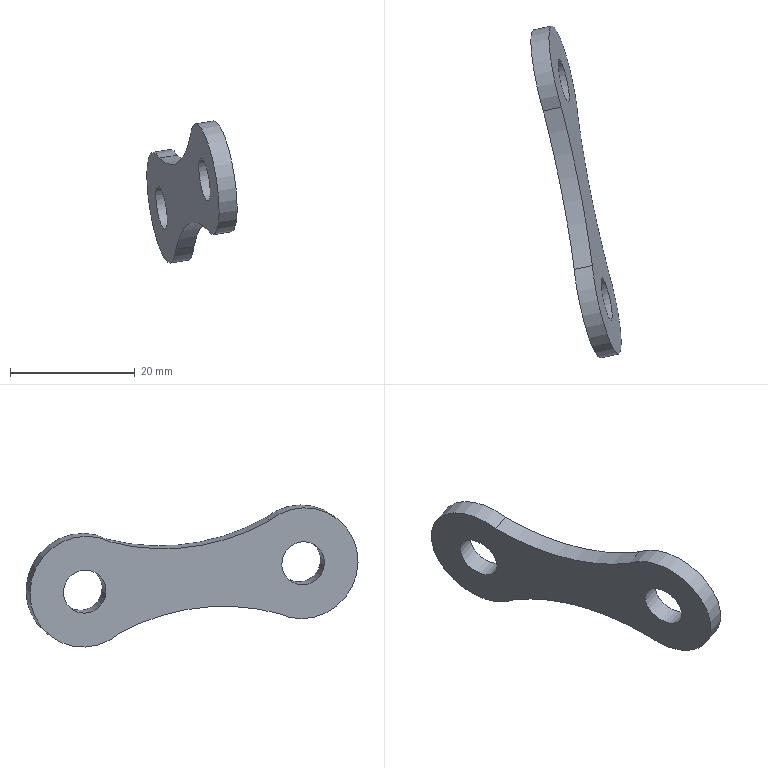Component | NX | 3_12 | 1 solid | 8 faces | box 14.49 x 53.27 x 22.8 mm | volume 1951 mm3 | cylinder 6 | plane 2 | commonest cylinder face diameters 70.075 x2 18 x2 7 x2
STEP:
#1=CARTESIAN_POINT('',(0.,0.,0.));
#2=DIRECTION('',(0.,0.,1.));
#3=DIRECTION('',(1.,0.,0.));
#4=AXIS2_PLACEMENT_3D('',#1,#2,#3);
#5=CARTESIAN_POINT('',(72.065,416.446,-165.474));
#6=VERTEX_POINT('',#5);
#7=CARTESIAN_POINT('',(74.96,417.076,-165.008));
#8=VERTEX_POINT('',#7);
#9=CARTESIAN_POINT('',(72.065,416.446,-165.474));
#10=DIRECTION('',(0.9653,0.21,0.1554));
#11=VECTOR('',#10,1.);
#12=LINE('',#9,#11);
#13=CARTESIAN_POINT('',(80.328,400.875,-195.754));
#14=DIRECTION('',(0.9653,0.21,0.1554));
#15=DIRECTION('',(0.1779,-0.09244,-0.9797));
#16=AXIS2_PLACEMENT_3D('',#13,#14,#15);
#17=CYLINDRICAL_SURFACE('',#16,35.038);
#18=CARTESIAN_POINT('',(2.764,-0.));
#19=DIRECTION('',(-0.,1.));
#20=VECTOR('',#19,1.);
#21=LINE('',#18,#20);
#22=(GEOMETRIC_REPRESENTATION_CONTEXT(2)PARAMETRIC_REPRESENTATION_CONTEXT()REPRESENTATION_CONTEXT('',''));
#23=DEFINITIONAL_REPRESENTATION('',(#21),#22);
#24=PCURVE('',#17,#23);
#25=CARTESIAN_POINT('',(69.774,422.032,-158.8));
#26=DIRECTION('',(0.9653,0.21,0.1554));
#27=DIRECTION('',(0.1779,-0.09244,-0.9797));
#28=AXIS2_PLACEMENT_3D('',#25,#26,#27);
#29=CYLINDRICAL_SURFACE('',#28,9.);
#30=CARTESIAN_POINT('',(-0.5931,-0.));
#31=DIRECTION('',(0.,1.));
#32=VECTOR('',#31,1.);
#33=LINE('',#30,#32);
#34=(GEOMETRIC_REPRESENTATION_CONTEXT(2)PARAMETRIC_REPRESENTATION_CONTEXT()REPRESENTATION_CONTEXT('',''));
#35=DEFINITIONAL_REPRESENTATION('',(#33),#34);
#36=PCURVE('',#29,#35);
#37=SURFACE_CURVE('',#12,(#24,#36),.PCURVE_S1.);
#38=EDGE_CURVE('',#6,#8,#37,.T.);
#39=ORIENTED_EDGE('',*,*,#38,.F.);
#40=CARTESIAN_POINT('',(77.093,390.984,-162.298));
#41=VERTEX_POINT('',#40);
#42=CARTESIAN_POINT('',(80.328,400.875,-195.754));
#43=DIRECTION('',(-0.9653,-0.21,-0.1554));
#44=DIRECTION('',(-0.1914,0.9733,-0.1266));
#45=AXIS2_PLACEMENT_3D('',#42,#43,#44);
#46=CIRCLE('',#45,35.038);
#47=CARTESIAN_POINT('',(7.854,0.));
#48=DIRECTION('',(-1.,-0.));
#49=VECTOR('',#48,1.);
#50=LINE('',#47,#49);
#51=(GEOMETRIC_REPRESENTATION_CONTEXT(2)PARAMETRIC_REPRESENTATION_CONTEXT()REPRESENTATION_CONTEXT('',''));
#52=DEFINITIONAL_REPRESENTATION('',(#50),#51);
#53=PCURVE('',#17,#52);
#54=CARTESIAN_POINT('',(75.051,411.454,-177.277));
#55=DIRECTION('',(-0.9653,-0.21,-0.1554));
#56=DIRECTION('',(-0.1779,0.09244,0.9797));
#57=AXIS2_PLACEMENT_3D('',#54,#55,#56);
#58=PLANE('',#57);
#59=CARTESIAN_POINT('',(-20.019,-8.967));
#60=DIRECTION('',(-0.,1.));
#61=AXIS2_PLACEMENT_2D('',#59,#60);
#62=CIRCLE('',#61,35.038);
#63=(GEOMETRIC_REPRESENTATION_CONTEXT(2)PARAMETRIC_REPRESENTATION_CONTEXT()REPRESENTATION_CONTEXT('',''));
#64=DEFINITIONAL_REPRESENTATION('',(#62),#63);
#65=PCURVE('',#58,#64);
#66=SURFACE_CURVE('',#46,(#53,#65),.PCURVE_S1.);
#67=EDGE_CURVE('',#41,#6,#66,.T.);
#68=ORIENTED_EDGE('',*,*,#67,.F.);
#69=CARTESIAN_POINT('',(79.988,391.614,-161.832));
#70=VERTEX_POINT('',#69);
#71=CARTESIAN_POINT('',(77.093,390.984,-162.298));
#72=DIRECTION('',(0.9653,0.21,0.1554));
#73=VECTOR('',#72,1.);
#74=LINE('',#71,#73);
#75=CARTESIAN_POINT('',(3.529,-0.));
#76=DIRECTION('',(0.,1.));
#77=VECTOR('',#76,1.);
#78=LINE('',#75,#77);
#79=(GEOMETRIC_REPRESENTATION_CONTEXT(2)PARAMETRIC_REPRESENTATION_CONTEXT()REPRESENTATION_CONTEXT('',''));
#80=DEFINITIONAL_REPRESENTATION('',(#78),#79);
#81=PCURVE('',#17,#80);
#82=CARTESIAN_POINT('',(76.664,386.993,-154.243));
#83=DIRECTION('',(0.9653,0.21,0.1554));
#84=DIRECTION('',(0.1779,-0.09244,-0.9797));
#85=AXIS2_PLACEMENT_3D('',#82,#83,#84);
#86=CYLINDRICAL_SURFACE('',#85,9.);
#87=CARTESIAN_POINT('',(6.849,-0.));
#88=DIRECTION('',(0.,1.));
#89=VECTOR('',#88,1.);
#90=LINE('',#87,#89);
#91=(GEOMETRIC_REPRESENTATION_CONTEXT(2)PARAMETRIC_REPRESENTATION_CONTEXT()REPRESENTATION_CONTEXT('',''));
#92=DEFINITIONAL_REPRESENTATION('',(#90),#91);
#93=PCURVE('',#86,#92);
#94=SURFACE_CURVE('',#74,(#81,#93),.PCURVE_S1.);
#95=EDGE_CURVE('',#41,#70,#94,.T.);
#96=ORIENTED_EDGE('',*,*,#95,.T.);
#97=CARTESIAN_POINT('',(83.224,401.505,-195.288));
#98=DIRECTION('',(-0.9653,-0.21,-0.1554));
#99=DIRECTION('',(-0.1914,0.9733,-0.1266));
#100=AXIS2_PLACEMENT_3D('',#97,#98,#99);
#101=CIRCLE('',#100,35.038);
#102=CARTESIAN_POINT('',(7.854,3.));
#103=DIRECTION('',(-1.,0.));
#104=VECTOR('',#103,1.);
#105=LINE('',#102,#104);
#106=(GEOMETRIC_REPRESENTATION_CONTEXT(2)PARAMETRIC_REPRESENTATION_CONTEXT()REPRESENTATION_CONTEXT('',''));
#107=DEFINITIONAL_REPRESENTATION('',(#105),#106);
#108=PCURVE('',#17,#107);
#109=CARTESIAN_POINT('',(77.947,412.084,-176.811));
#110=DIRECTION('',(-0.9653,-0.21,-0.1554));
#111=DIRECTION('',(-0.1779,0.09244,0.9797));
#112=AXIS2_PLACEMENT_3D('',#109,#110,#111);
#113=PLANE('',#112);
#114=CARTESIAN_POINT('',(-20.019,-8.967));
#115=DIRECTION('',(-0.,1.));
#116=AXIS2_PLACEMENT_2D('',#114,#115);
#117=CIRCLE('',#116,35.038);
#118=(GEOMETRIC_REPRESENTATION_CONTEXT(2)PARAMETRIC_REPRESENTATION_CONTEXT()REPRESENTATION_CONTEXT('',''));
#119=DEFINITIONAL_REPRESENTATION('',(#117),#118);
#120=PCURVE('',#113,#119);
#121=SURFACE_CURVE('',#101,(#108,#120),.PCURVE_S1.);
#122=EDGE_CURVE('',#70,#8,#121,.T.);
#123=ORIENTED_EDGE('',*,*,#122,.T.);
#124=EDGE_LOOP('',(#39,#68,#96,#123));
#125=FACE_BOUND('',#124,.F.);
#126=ADVANCED_FACE('',(#125),#17,.F.);
#127=CARTESIAN_POINT('',(72.306,418.456,-150.385));
#128=VERTEX_POINT('',#127);
#129=CARTESIAN_POINT('',(72.67,422.662,-158.333));
#130=DIRECTION('',(0.9653,0.21,0.1554));
#131=DIRECTION('',(-0.1914,0.9733,-0.1266));
#132=AXIS2_PLACEMENT_3D('',#129,#130,#131);
#133=CIRCLE('',#132,9.);
#134=CARTESIAN_POINT('',(-4.712,3.));
#135=DIRECTION('',(1.,0.));
#136=VECTOR('',#135,1.);
#137=LINE('',#134,#136);
#138=(GEOMETRIC_REPRESENTATION_CONTEXT(2)PARAMETRIC_REPRESENTATION_CONTEXT()REPRESENTATION_CONTEXT('',''));
#139=DEFINITIONAL_REPRESENTATION('',(#137),#138);
#140=PCURVE('',#29,#139);
#141=CARTESIAN_POINT('',(20.019,17.967));
#142=CARTESIAN_POINT('',(35.607,17.967));
#143=CARTESIAN_POINT('',(27.813,4.467));
#144=CARTESIAN_POINT('',(20.019,-9.033));
#145=CARTESIAN_POINT('',(12.225,4.467));
#146=CARTESIAN_POINT('',(4.43,17.967));
#147=CARTESIAN_POINT('',(20.019,17.967));
#148=(BOUNDED_CURVE()B_SPLINE_CURVE(2,(#141,#142,#143,#144,#145,#146,#147),.UNSPECIFIED.,.T.,.F.)B_SPLINE_CURVE_WITH_KNOTS((1,2,2,2,2,1),(-2.094,0.,2.094,4.189,6.283,8.378),.UNSPECIFIED.)CURVE()GEOMETRIC_REPRESENTATION_ITEM()RATIONAL_B_SPLINE_CURVE((1.,0.5,1.,0.5,1.,0.5,1.))REPRESENTATION_ITEM(''));
#149=(GEOMETRIC_REPRESENTATION_CONTEXT(2)PARAMETRIC_REPRESENTATION_CONTEXT()REPRESENTATION_CONTEXT('',''));
#150=DEFINITIONAL_REPRESENTATION('',(#148),#149);
#151=PCURVE('',#113,#150);
#152=SURFACE_CURVE('',#133,(#140,#151),.PCURVE_S1.);
#153=EDGE_CURVE('',#8,#128,#152,.T.);
#154=ORIENTED_EDGE('',*,*,#153,.F.);
#155=ORIENTED_EDGE('',*,*,#38,.F.);
#156=CARTESIAN_POINT('',(69.41,417.826,-150.852));
#157=VERTEX_POINT('',#156);
#158=CARTESIAN_POINT('',(69.774,422.032,-158.8));
#159=DIRECTION('',(0.9653,0.21,0.1554));
#160=DIRECTION('',(-0.1914,0.9733,-0.1266));
#161=AXIS2_PLACEMENT_3D('',#158,#159,#160);
#162=CIRCLE('',#161,9.);
#163=CARTESIAN_POINT('',(-4.712,-0.));
#164=DIRECTION('',(1.,0.));
#165=VECTOR('',#164,1.);
#166=LINE('',#163,#165);
#167=(GEOMETRIC_REPRESENTATION_CONTEXT(2)PARAMETRIC_REPRESENTATION_CONTEXT()REPRESENTATION_CONTEXT('',''));
#168=DEFINITIONAL_REPRESENTATION('',(#166),#167);
#169=PCURVE('',#29,#168);
#170=CARTESIAN_POINT('',(20.019,17.967));
#171=CARTESIAN_POINT('',(35.607,17.967));
#172=CARTESIAN_POINT('',(27.813,4.467));
#173=CARTESIAN_POINT('',(20.019,-9.033));
#174=CARTESIAN_POINT('',(12.225,4.467));
#175=CARTESIAN_POINT('',(4.43,17.967));
#176=CARTESIAN_POINT('',(20.019,17.967));
#177=(BOUNDED_CURVE()B_SPLINE_CURVE(2,(#170,#171,#172,#173,#174,#175,#176),.UNSPECIFIED.,.T.,.F.)B_SPLINE_CURVE_WITH_KNOTS((1,2,2,2,2,1),(-2.094,0.,2.094,4.189,6.283,8.378),.UNSPECIFIED.)CURVE()GEOMETRIC_REPRESENTATION_ITEM()RATIONAL_B_SPLINE_CURVE((1.,0.5,1.,0.5,1.,0.5,1.))REPRESENTATION_ITEM(''));
#178=(GEOMETRIC_REPRESENTATION_CONTEXT(2)PARAMETRIC_REPRESENTATION_CONTEXT()REPRESENTATION_CONTEXT('',''));
#179=DEFINITIONAL_REPRESENTATION('',(#177),#178);
#180=PCURVE('',#58,#179);
#181=SURFACE_CURVE('',#162,(#169,#180),.PCURVE_S1.);
#182=EDGE_CURVE('',#6,#157,#181,.T.);
#183=ORIENTED_EDGE('',*,*,#182,.T.);
#184=CARTESIAN_POINT('',(69.41,417.826,-150.852));
#185=DIRECTION('',(0.9653,0.21,0.1554));
#186=VECTOR('',#185,1.);
#187=LINE('',#184,#186);
#188=CARTESIAN_POINT('',(3.735,0.));
#189=DIRECTION('',(-0.,1.));
#190=VECTOR('',#189,1.);
#191=LINE('',#188,#190);
#192=(GEOMETRIC_REPRESENTATION_CONTEXT(2)PARAMETRIC_REPRESENTATION_CONTEXT()REPRESENTATION_CONTEXT('',''));
#193=DEFINITIONAL_REPRESENTATION('',(#191),#192);
#194=PCURVE('',#29,#193);
#195=CARTESIAN_POINT('',(66.085,408.277,-117.305));
#196=DIRECTION('',(0.9653,0.21,0.1554));
#197=DIRECTION('',(0.1779,-0.09244,-0.9797));
#198=AXIS2_PLACEMENT_3D('',#195,#196,#197);
#199=CYLINDRICAL_SURFACE('',#198,35.038);
#200=CARTESIAN_POINT('',(6.66,0.));
#201=DIRECTION('',(0.,1.));
#202=VECTOR('',#201,1.);
#203=LINE('',#200,#202);
#204=(GEOMETRIC_REPRESENTATION_CONTEXT(2)PARAMETRIC_REPRESENTATION_CONTEXT()REPRESENTATION_CONTEXT('',''));
#205=DEFINITIONAL_REPRESENTATION('',(#203),#204);
#206=PCURVE('',#199,#205);
#207=SURFACE_CURVE('',#187,(#194,#206),.PCURVE_S1.);
#208=EDGE_CURVE('',#157,#128,#207,.T.);
#209=ORIENTED_EDGE('',*,*,#208,.T.);
#210=EDGE_LOOP('',(#154,#155,#183,#209));
#211=FACE_BOUND('',#210,.T.);
#212=ADVANCED_FACE('',(#211),#29,.T.);
#213=CARTESIAN_POINT('',(74.389,392.389,-147.408));
#214=VERTEX_POINT('',#213);
#215=CARTESIAN_POINT('',(77.285,393.019,-146.942));
#216=VERTEX_POINT('',#215);
#217=CARTESIAN_POINT('',(74.389,392.389,-147.408));
#218=DIRECTION('',(0.9653,0.21,0.1554));
#219=VECTOR('',#218,1.);
#220=LINE('',#217,#219);
#221=CARTESIAN_POINT('',(5.896,0.));
#222=DIRECTION('',(0.,1.));
#223=VECTOR('',#222,1.);
#224=LINE('',#221,#223);
#225=(GEOMETRIC_REPRESENTATION_CONTEXT(2)PARAMETRIC_REPRESENTATION_CONTEXT()REPRESENTATION_CONTEXT('',''));
#226=DEFINITIONAL_REPRESENTATION('',(#224),#225);
#227=PCURVE('',#199,#226);
#228=CARTESIAN_POINT('',(2.576,-0.));
#229=DIRECTION('',(0.,1.));
#230=VECTOR('',#229,1.);
#231=LINE('',#228,#230);
#232=(GEOMETRIC_REPRESENTATION_CONTEXT(2)PARAMETRIC_REPRESENTATION_CONTEXT()REPRESENTATION_CONTEXT('',''));
#233=DEFINITIONAL_REPRESENTATION('',(#231),#232);
#234=PCURVE('',#86,#233);
#235=SURFACE_CURVE('',#220,(#227,#234),.PCURVE_S1.);
#236=EDGE_CURVE('',#214,#216,#235,.T.);
#237=ORIENTED_EDGE('',*,*,#236,.F.);
#238=CARTESIAN_POINT('',(66.085,408.277,-117.305));
#239=DIRECTION('',(-0.9653,-0.21,-0.1554));
#240=DIRECTION('',(-0.1914,0.9733,-0.1266));
#241=AXIS2_PLACEMENT_3D('',#238,#239,#240);
#242=CIRCLE('',#241,35.038);
#243=CARTESIAN_POINT('',(7.854,0.));
#244=DIRECTION('',(-1.,0.));
#245=VECTOR('',#244,1.);
#246=LINE('',#243,#245);
#247=(GEOMETRIC_REPRESENTATION_CONTEXT(2)PARAMETRIC_REPRESENTATION_CONTEXT()REPRESENTATION_CONTEXT('',''));
#248=DEFINITIONAL_REPRESENTATION('',(#246),#247);
#249=PCURVE('',#199,#248);
#250=CARTESIAN_POINT('',(60.056,-8.967));
#251=DIRECTION('',(-0.,1.));
#252=AXIS2_PLACEMENT_2D('',#250,#251);
#253=CIRCLE('',#252,35.038);
#254=(GEOMETRIC_REPRESENTATION_CONTEXT(2)PARAMETRIC_REPRESENTATION_CONTEXT()REPRESENTATION_CONTEXT('',''));
#255=DEFINITIONAL_REPRESENTATION('',(#253),#254);
#256=PCURVE('',#58,#255);
#257=SURFACE_CURVE('',#242,(#249,#256),.PCURVE_S1.);
#258=EDGE_CURVE('',#157,#214,#257,.T.);
#259=ORIENTED_EDGE('',*,*,#258,.F.);
#260=ORIENTED_EDGE('',*,*,#208,.T.);
#261=CARTESIAN_POINT('',(68.981,408.907,-116.838));
#262=DIRECTION('',(-0.9653,-0.21,-0.1554));
#263=DIRECTION('',(-0.1914,0.9733,-0.1266));
#264=AXIS2_PLACEMENT_3D('',#261,#262,#263);
#265=CIRCLE('',#264,35.038);
#266=CARTESIAN_POINT('',(7.854,3.));
#267=DIRECTION('',(-1.,0.));
#268=VECTOR('',#267,1.);
#269=LINE('',#266,#268);
#270=(GEOMETRIC_REPRESENTATION_CONTEXT(2)PARAMETRIC_REPRESENTATION_CONTEXT()REPRESENTATION_CONTEXT('',''));
#271=DEFINITIONAL_REPRESENTATION('',(#269),#270);
#272=PCURVE('',#199,#271);
#273=CARTESIAN_POINT('',(60.056,-8.967));
#274=DIRECTION('',(-0.,1.));
#275=AXIS2_PLACEMENT_2D('',#273,#274);
#276=CIRCLE('',#275,35.038);
#277=(GEOMETRIC_REPRESENTATION_CONTEXT(2)PARAMETRIC_REPRESENTATION_CONTEXT()REPRESENTATION_CONTEXT('',''));
#278=DEFINITIONAL_REPRESENTATION('',(#276),#277);
#279=PCURVE('',#113,#278);
#280=SURFACE_CURVE('',#265,(#272,#279),.PCURVE_S1.);
#281=EDGE_CURVE('',#128,#216,#280,.T.);
#282=ORIENTED_EDGE('',*,*,#281,.T.);
#283=EDGE_LOOP('',(#237,#259,#260,#282));
#284=FACE_BOUND('',#283,.F.);
#285=ADVANCED_FACE('',(#284),#199,.F.);
#286=CARTESIAN_POINT('',(75.994,390.399,-154.686));
#287=VERTEX_POINT('',#286);
#288=CARTESIAN_POINT('',(76.664,386.993,-154.243));
#289=DIRECTION('',(0.9653,0.21,0.1554));
#290=DIRECTION('',(-0.1914,0.9733,-0.1266));
#291=AXIS2_PLACEMENT_3D('',#288,#289,#290);
#292=CIRCLE('',#291,3.5);
#293=CARTESIAN_POINT('',(76.664,386.993,-154.243));
#294=DIRECTION('',(0.9653,0.21,0.1554));
#295=DIRECTION('',(0.1779,-0.09244,-0.9797));
#296=AXIS2_PLACEMENT_3D('',#293,#294,#295);
#297=CYLINDRICAL_SURFACE('',#296,3.5);
#298=CARTESIAN_POINT('',(1.571,0.));
#299=DIRECTION('',(1.,0.));
#300=VECTOR('',#299,1.);
#301=LINE('',#298,#300);
#302=(GEOMETRIC_REPRESENTATION_CONTEXT(2)PARAMETRIC_REPRESENTATION_CONTEXT()REPRESENTATION_CONTEXT('',''));
#303=DEFINITIONAL_REPRESENTATION('',(#301),#302);
#304=PCURVE('',#297,#303);
#305=CARTESIAN_POINT('',(20.019,-23.533));
#306=CARTESIAN_POINT('',(26.081,-23.533));
#307=CARTESIAN_POINT('',(23.05,-28.783));
#308=CARTESIAN_POINT('',(20.019,-34.033));
#309=CARTESIAN_POINT('',(16.988,-28.783));
#310=CARTESIAN_POINT('',(13.957,-23.533));
#311=CARTESIAN_POINT('',(20.019,-23.533));
#312=(BOUNDED_CURVE()B_SPLINE_CURVE(2,(#305,#306,#307,#308,#309,#310,#311),.UNSPECIFIED.,.T.,.F.)B_SPLINE_CURVE_WITH_KNOTS((1,2,2,2,2,1),(-2.094,0.,2.094,4.189,6.283,8.378),.UNSPECIFIED.)CURVE()GEOMETRIC_REPRESENTATION_ITEM()RATIONAL_B_SPLINE_CURVE((1.,0.5,1.,0.5,1.,0.5,1.))REPRESENTATION_ITEM(''));
#313=(GEOMETRIC_REPRESENTATION_CONTEXT(2)PARAMETRIC_REPRESENTATION_CONTEXT()REPRESENTATION_CONTEXT('',''));
#314=DEFINITIONAL_REPRESENTATION('',(#312),#313);
#315=PCURVE('',#58,#314);
#316=SURFACE_CURVE('',#292,(#304,#315),.PCURVE_S1.);
#317=EDGE_CURVE('',#287,#287,#316,.T.);
#318=ORIENTED_EDGE('',*,*,#317,.T.);
#319=CARTESIAN_POINT('',(78.89,391.029,-154.219));
#320=VERTEX_POINT('',#319);
#321=CARTESIAN_POINT('',(75.994,390.399,-154.686));
#322=CARTESIAN_POINT('',(78.89,391.029,-154.219));
#323=B_SPLINE_CURVE_WITH_KNOTS('',1,(#321,#322),.UNSPECIFIED.,.F.,.F.,(2,2),(0.,3.),.PIECEWISE_BEZIER_KNOTS.);
#324=CARTESIAN_POINT('',(7.854,0.));
#325=DIRECTION('',(0.,1.));
#326=VECTOR('',#325,1.);
#327=LINE('',#324,#326);
#328=(GEOMETRIC_REPRESENTATION_CONTEXT(2)PARAMETRIC_REPRESENTATION_CONTEXT()REPRESENTATION_CONTEXT('',''));
#329=DEFINITIONAL_REPRESENTATION('',(#327),#328);
#330=PCURVE('',#297,#329);
#331=CARTESIAN_POINT('',(1.571,0.));
#332=DIRECTION('',(0.,1.));
#333=VECTOR('',#332,1.);
#334=LINE('',#331,#333);
#335=(GEOMETRIC_REPRESENTATION_CONTEXT(2)PARAMETRIC_REPRESENTATION_CONTEXT()REPRESENTATION_CONTEXT('',''));
#336=DEFINITIONAL_REPRESENTATION('',(#334),#335);
#337=PCURVE('',#297,#336);
#338=SEAM_CURVE('',#323,(#330,#337),.PCURVE_S1.);
#339=EDGE_CURVE('',#287,#320,#338,.T.);
#340=ORIENTED_EDGE('',*,*,#339,.T.);
#341=CARTESIAN_POINT('',(79.56,387.623,-153.776));
#342=DIRECTION('',(0.9653,0.21,0.1554));
#343=DIRECTION('',(-0.1914,0.9733,-0.1266));
#344=AXIS2_PLACEMENT_3D('',#341,#342,#343);
#345=CIRCLE('',#344,3.5);
#346=CARTESIAN_POINT('',(1.571,3.));
#347=DIRECTION('',(1.,0.));
#348=VECTOR('',#347,1.);
#349=LINE('',#346,#348);
#350=(GEOMETRIC_REPRESENTATION_CONTEXT(2)PARAMETRIC_REPRESENTATION_CONTEXT()REPRESENTATION_CONTEXT('',''));
#351=DEFINITIONAL_REPRESENTATION('',(#349),#350);
#352=PCURVE('',#297,#351);
#353=CARTESIAN_POINT('',(20.019,-23.533));
#354=CARTESIAN_POINT('',(26.081,-23.533));
#355=CARTESIAN_POINT('',(23.05,-28.783));
#356=CARTESIAN_POINT('',(20.019,-34.033));
#357=CARTESIAN_POINT('',(16.988,-28.783));
#358=CARTESIAN_POINT('',(13.957,-23.533));
#359=CARTESIAN_POINT('',(20.019,-23.533));
#360=(BOUNDED_CURVE()B_SPLINE_CURVE(2,(#353,#354,#355,#356,#357,#358,#359),.UNSPECIFIED.,.T.,.F.)B_SPLINE_CURVE_WITH_KNOTS((1,2,2,2,2,1),(-2.094,0.,2.094,4.189,6.283,8.378),.UNSPECIFIED.)CURVE()GEOMETRIC_REPRESENTATION_ITEM()RATIONAL_B_SPLINE_CURVE((1.,0.5,1.,0.5,1.,0.5,1.))REPRESENTATION_ITEM(''));
#361=(GEOMETRIC_REPRESENTATION_CONTEXT(2)PARAMETRIC_REPRESENTATION_CONTEXT()REPRESENTATION_CONTEXT('',''));
#362=DEFINITIONAL_REPRESENTATION('',(#360),#361);
#363=PCURVE('',#113,#362);
#364=SURFACE_CURVE('',#345,(#352,#363),.PCURVE_S1.);
#365=EDGE_CURVE('',#320,#320,#364,.T.);
#366=ORIENTED_EDGE('',*,*,#365,.F.);
#367=ORIENTED_EDGE('',*,*,#339,.F.);
#368=EDGE_LOOP('',(#318,#340,#366,#367));
#369=FACE_BOUND('',#368,.F.);
#370=ADVANCED_FACE('',(#369),#297,.F.);
#371=CARTESIAN_POINT('',(79.56,387.623,-153.776));
#372=DIRECTION('',(0.9653,0.21,0.1554));
#373=DIRECTION('',(-0.1914,0.9733,-0.1266));
#374=AXIS2_PLACEMENT_3D('',#371,#372,#373);
#375=CIRCLE('',#374,9.);
#376=CARTESIAN_POINT('',(1.571,3.));
#377=DIRECTION('',(1.,-0.));
#378=VECTOR('',#377,1.);
#379=LINE('',#376,#378);
#380=(GEOMETRIC_REPRESENTATION_CONTEXT(2)PARAMETRIC_REPRESENTATION_CONTEXT()REPRESENTATION_CONTEXT('',''));
#381=DEFINITIONAL_REPRESENTATION('',(#379),#380);
#382=PCURVE('',#86,#381);
#383=CARTESIAN_POINT('',(20.019,-18.033));
#384=CARTESIAN_POINT('',(35.607,-18.033));
#385=CARTESIAN_POINT('',(27.813,-31.533));
#386=CARTESIAN_POINT('',(20.019,-45.033));
#387=CARTESIAN_POINT('',(12.225,-31.533));
#388=CARTESIAN_POINT('',(4.43,-18.033));
#389=CARTESIAN_POINT('',(20.019,-18.033));
#390=(BOUNDED_CURVE()B_SPLINE_CURVE(2,(#383,#384,#385,#386,#387,#388,#389),.UNSPECIFIED.,.T.,.F.)B_SPLINE_CURVE_WITH_KNOTS((1,2,2,2,2,1),(-2.094,0.,2.094,4.189,6.283,8.378),.UNSPECIFIED.)CURVE()GEOMETRIC_REPRESENTATION_ITEM()RATIONAL_B_SPLINE_CURVE((1.,0.5,1.,0.5,1.,0.5,1.))REPRESENTATION_ITEM(''));
#391=(GEOMETRIC_REPRESENTATION_CONTEXT(2)PARAMETRIC_REPRESENTATION_CONTEXT()REPRESENTATION_CONTEXT('',''));
#392=DEFINITIONAL_REPRESENTATION('',(#390),#391);
#393=PCURVE('',#113,#392);
#394=SURFACE_CURVE('',#375,(#382,#393),.PCURVE_S1.);
#395=EDGE_CURVE('',#216,#70,#394,.T.);
#396=ORIENTED_EDGE('',*,*,#395,.F.);
#397=ORIENTED_EDGE('',*,*,#236,.F.);
#398=CARTESIAN_POINT('',(76.664,386.993,-154.243));
#399=DIRECTION('',(0.9653,0.21,0.1554));
#400=DIRECTION('',(-0.1914,0.9733,-0.1266));
#401=AXIS2_PLACEMENT_3D('',#398,#399,#400);
#402=CIRCLE('',#401,9.);
#403=CARTESIAN_POINT('',(1.571,-0.));
#404=DIRECTION('',(1.,0.));
#405=VECTOR('',#404,1.);
#406=LINE('',#403,#405);
#407=(GEOMETRIC_REPRESENTATION_CONTEXT(2)PARAMETRIC_REPRESENTATION_CONTEXT()REPRESENTATION_CONTEXT('',''));
#408=DEFINITIONAL_REPRESENTATION('',(#406),#407);
#409=PCURVE('',#86,#408);
#410=CARTESIAN_POINT('',(20.019,-18.033));
#411=CARTESIAN_POINT('',(35.607,-18.033));
#412=CARTESIAN_POINT('',(27.813,-31.533));
#413=CARTESIAN_POINT('',(20.019,-45.033));
#414=CARTESIAN_POINT('',(12.225,-31.533));
#415=CARTESIAN_POINT('',(4.43,-18.033));
#416=CARTESIAN_POINT('',(20.019,-18.033));
#417=(BOUNDED_CURVE()B_SPLINE_CURVE(2,(#410,#411,#412,#413,#414,#415,#416),.UNSPECIFIED.,.T.,.F.)B_SPLINE_CURVE_WITH_KNOTS((1,2,2,2,2,1),(-2.094,0.,2.094,4.189,6.283,8.378),.UNSPECIFIED.)CURVE()GEOMETRIC_REPRESENTATION_ITEM()RATIONAL_B_SPLINE_CURVE((1.,0.5,1.,0.5,1.,0.5,1.))REPRESENTATION_ITEM(''));
#418=(GEOMETRIC_REPRESENTATION_CONTEXT(2)PARAMETRIC_REPRESENTATION_CONTEXT()REPRESENTATION_CONTEXT('',''));
#419=DEFINITIONAL_REPRESENTATION('',(#417),#418);
#420=PCURVE('',#58,#419);
#421=SURFACE_CURVE('',#402,(#409,#420),.PCURVE_S1.);
#422=EDGE_CURVE('',#214,#41,#421,.T.);
#423=ORIENTED_EDGE('',*,*,#422,.T.);
#424=ORIENTED_EDGE('',*,*,#95,.T.);
#425=EDGE_LOOP('',(#396,#397,#423,#424));
#426=FACE_BOUND('',#425,.T.);
#427=ADVANCED_FACE('',(#426),#86,.T.);
#428=CARTESIAN_POINT('',(69.105,425.439,-159.243));
#429=VERTEX_POINT('',#428);
#430=CARTESIAN_POINT('',(69.774,422.032,-158.8));
#431=DIRECTION('',(0.9653,0.21,0.1554));
#432=DIRECTION('',(-0.1914,0.9733,-0.1266));
#433=AXIS2_PLACEMENT_3D('',#430,#431,#432);
#434=CIRCLE('',#433,3.5);
#435=CARTESIAN_POINT('',(69.774,422.032,-158.8));
#436=DIRECTION('',(0.9653,0.21,0.1554));
#437=DIRECTION('',(0.1779,-0.09244,-0.9797));
#438=AXIS2_PLACEMENT_3D('',#435,#436,#437);
#439=CYLINDRICAL_SURFACE('',#438,3.5);
#440=CARTESIAN_POINT('',(1.571,0.));
#441=DIRECTION('',(1.,0.));
#442=VECTOR('',#441,1.);
#443=LINE('',#440,#442);
#444=(GEOMETRIC_REPRESENTATION_CONTEXT(2)PARAMETRIC_REPRESENTATION_CONTEXT()REPRESENTATION_CONTEXT('',''));
#445=DEFINITIONAL_REPRESENTATION('',(#443),#444);
#446=PCURVE('',#439,#445);
#447=CARTESIAN_POINT('',(20.019,12.467));
#448=CARTESIAN_POINT('',(26.081,12.467));
#449=CARTESIAN_POINT('',(23.05,7.217));
#450=CARTESIAN_POINT('',(20.019,1.967));
#451=CARTESIAN_POINT('',(16.988,7.217));
#452=CARTESIAN_POINT('',(13.957,12.467));
#453=CARTESIAN_POINT('',(20.019,12.467));
#454=(BOUNDED_CURVE()B_SPLINE_CURVE(2,(#447,#448,#449,#450,#451,#452,#453),.UNSPECIFIED.,.T.,.F.)B_SPLINE_CURVE_WITH_KNOTS((1,2,2,2,2,1),(-2.094,0.,2.094,4.189,6.283,8.378),.UNSPECIFIED.)CURVE()GEOMETRIC_REPRESENTATION_ITEM()RATIONAL_B_SPLINE_CURVE((1.,0.5,1.,0.5,1.,0.5,1.))REPRESENTATION_ITEM(''));
#455=(GEOMETRIC_REPRESENTATION_CONTEXT(2)PARAMETRIC_REPRESENTATION_CONTEXT()REPRESENTATION_CONTEXT('',''));
#456=DEFINITIONAL_REPRESENTATION('',(#454),#455);
#457=PCURVE('',#58,#456);
#458=SURFACE_CURVE('',#434,(#446,#457),.PCURVE_S1.);
#459=EDGE_CURVE('',#429,#429,#458,.T.);
#460=ORIENTED_EDGE('',*,*,#459,.T.);
#461=CARTESIAN_POINT('',(72.,426.069,-158.776));
#462=VERTEX_POINT('',#461);
#463=CARTESIAN_POINT('',(69.105,425.439,-159.243));
#464=CARTESIAN_POINT('',(72.,426.069,-158.776));
#465=B_SPLINE_CURVE_WITH_KNOTS('',1,(#463,#464),.UNSPECIFIED.,.F.,.F.,(2,2),(0.,3.),.PIECEWISE_BEZIER_KNOTS.);
#466=CARTESIAN_POINT('',(7.854,0.));
#467=DIRECTION('',(0.,1.));
#468=VECTOR('',#467,1.);
#469=LINE('',#466,#468);
#470=(GEOMETRIC_REPRESENTATION_CONTEXT(2)PARAMETRIC_REPRESENTATION_CONTEXT()REPRESENTATION_CONTEXT('',''));
#471=DEFINITIONAL_REPRESENTATION('',(#469),#470);
#472=PCURVE('',#439,#471);
#473=CARTESIAN_POINT('',(1.571,0.));
#474=DIRECTION('',(0.,1.));
#475=VECTOR('',#474,1.);
#476=LINE('',#473,#475);
#477=(GEOMETRIC_REPRESENTATION_CONTEXT(2)PARAMETRIC_REPRESENTATION_CONTEXT()REPRESENTATION_CONTEXT('',''));
#478=DEFINITIONAL_REPRESENTATION('',(#476),#477);
#479=PCURVE('',#439,#478);
#480=SEAM_CURVE('',#465,(#472,#479),.PCURVE_S1.);
#481=EDGE_CURVE('',#429,#462,#480,.T.);
#482=ORIENTED_EDGE('',*,*,#481,.T.);
#483=CARTESIAN_POINT('',(72.67,422.662,-158.333));
#484=DIRECTION('',(0.9653,0.21,0.1554));
#485=DIRECTION('',(-0.1914,0.9733,-0.1266));
#486=AXIS2_PLACEMENT_3D('',#483,#484,#485);
#487=CIRCLE('',#486,3.5);
#488=CARTESIAN_POINT('',(1.571,3.));
#489=DIRECTION('',(1.,0.));
#490=VECTOR('',#489,1.);
#491=LINE('',#488,#490);
#492=(GEOMETRIC_REPRESENTATION_CONTEXT(2)PARAMETRIC_REPRESENTATION_CONTEXT()REPRESENTATION_CONTEXT('',''));
#493=DEFINITIONAL_REPRESENTATION('',(#491),#492);
#494=PCURVE('',#439,#493);
#495=CARTESIAN_POINT('',(20.019,12.467));
#496=CARTESIAN_POINT('',(26.081,12.467));
#497=CARTESIAN_POINT('',(23.05,7.217));
#498=CARTESIAN_POINT('',(20.019,1.967));
#499=CARTESIAN_POINT('',(16.988,7.217));
#500=CARTESIAN_POINT('',(13.957,12.467));
#501=CARTESIAN_POINT('',(20.019,12.467));
#502=(BOUNDED_CURVE()B_SPLINE_CURVE(2,(#495,#496,#497,#498,#499,#500,#501),.UNSPECIFIED.,.T.,.F.)B_SPLINE_CURVE_WITH_KNOTS((1,2,2,2,2,1),(-2.094,0.,2.094,4.189,6.283,8.378),.UNSPECIFIED.)CURVE()GEOMETRIC_REPRESENTATION_ITEM()RATIONAL_B_SPLINE_CURVE((1.,0.5,1.,0.5,1.,0.5,1.))REPRESENTATION_ITEM(''));
#503=(GEOMETRIC_REPRESENTATION_CONTEXT(2)PARAMETRIC_REPRESENTATION_CONTEXT()REPRESENTATION_CONTEXT('',''));
#504=DEFINITIONAL_REPRESENTATION('',(#502),#503);
#505=PCURVE('',#113,#504);
#506=SURFACE_CURVE('',#487,(#494,#505),.PCURVE_S1.);
#507=EDGE_CURVE('',#462,#462,#506,.T.);
#508=ORIENTED_EDGE('',*,*,#507,.F.);
#509=ORIENTED_EDGE('',*,*,#481,.F.);
#510=EDGE_LOOP('',(#460,#482,#508,#509));
#511=FACE_BOUND('',#510,.F.);
#512=ADVANCED_FACE('',(#511),#439,.F.);
#513=ORIENTED_EDGE('',*,*,#67,.F.);
#514=ORIENTED_EDGE('',*,*,#422,.F.);
#515=ORIENTED_EDGE('',*,*,#258,.F.);
#516=ORIENTED_EDGE('',*,*,#182,.F.);
#517=EDGE_LOOP('',(#513,#514,#515,#516));
#518=FACE_BOUND('',#517,.T.);
#519=ORIENTED_EDGE('',*,*,#317,.T.);
#520=EDGE_LOOP('',(#519));
#521=FACE_BOUND('',#520,.T.);
#522=ORIENTED_EDGE('',*,*,#459,.T.);
#523=EDGE_LOOP('',(#522));
#524=FACE_BOUND('',#523,.T.);
#525=ADVANCED_FACE('',(#518,#521,#524),#58,.T.);
#526=ORIENTED_EDGE('',*,*,#122,.T.);
#527=ORIENTED_EDGE('',*,*,#153,.T.);
#528=ORIENTED_EDGE('',*,*,#281,.T.);
#529=ORIENTED_EDGE('',*,*,#395,.T.);
#530=EDGE_LOOP('',(#526,#527,#528,#529));
#531=FACE_BOUND('',#530,.T.);
#532=ORIENTED_EDGE('',*,*,#365,.F.);
#533=EDGE_LOOP('',(#532));
#534=FACE_BOUND('',#533,.T.);
#535=ORIENTED_EDGE('',*,*,#507,.F.);
#536=EDGE_LOOP('',(#535));
#537=FACE_BOUND('',#536,.T.);
#538=ADVANCED_FACE('',(#531,#534,#537),#113,.F.);
#539=CLOSED_SHELL('',(#126,#212,#285,#370,#427,#512,#525,#538));
#540=MANIFOLD_SOLID_BREP('',#539);
#541=(LENGTH_UNIT()NAMED_UNIT(*)SI_UNIT(.MILLI.,.METRE.));
#542=UNCERTAINTY_MEASURE_WITH_UNIT(LENGTH_MEASURE(0.000002),#541,'','');
#543=(NAMED_UNIT(*)PLANE_ANGLE_UNIT()SI_UNIT($,.RADIAN.));
#544=(NAMED_UNIT(*)SI_UNIT($,.STERADIAN.)SOLID_ANGLE_UNIT());
#545=(GEOMETRIC_REPRESENTATION_CONTEXT(3)GLOBAL_UNCERTAINTY_ASSIGNED_CONTEXT((#542))GLOBAL_UNIT_ASSIGNED_CONTEXT((#541,#543,#544))REPRESENTATION_CONTEXT('',''));
#546=ADVANCED_BREP_SHAPE_REPRESENTATION('',(#4,#540),#545);